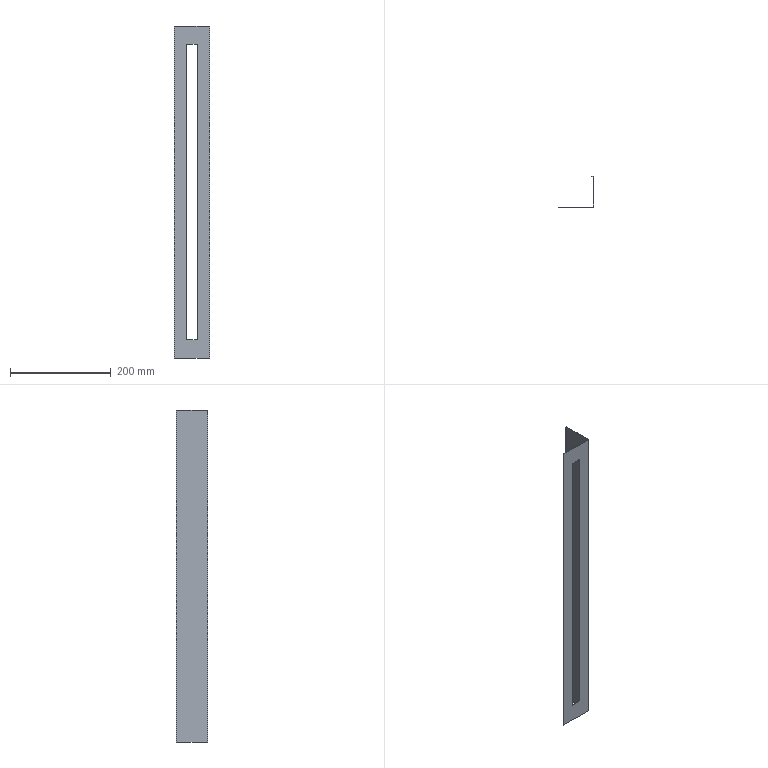Component | SolidWorks | MotorCover-1 | 1 solid | 16 faces | box 70 x 62 x 660 mm | volume 37993 mm3 | plane 14 | cylinder 2 | commonest cylinder face diameters 1 x2
build123d program:
from build123d import *

# Parameters (mm, degrees)
BOSS_EXTRUDE1_DEPTH = 660
SKETCH2_W           = 588
SKETCH2_H           = 21.5
CUT_EXTRUDE1_DEPTH  = 10


with BuildPart() as part:
    # Sketch1 → Boss-Extrude1 (new body)
    with BuildSketch(Plane.XY):
        with BuildLine():
            Line((0, 0), (0, 69.5))
            ThreePointArc((0, 69.5), (0.1464, 69.854), (0.5, 70))
            Line((0.5, 70), (61.5, 70))
            ThreePointArc((61.5, 70), (61.854, 69.854), (62, 69.5))
            Line((62, 69.5), (62, 66.5))
            Line((62, 66.5), (61.5, 66.5))
            Line((61.5, 66.5), (61.5, 69.5))
            Line((61.5, 69.5), (0.5, 69.5))
            Line((0.5, 69.5), (0.5, 0))
            Line((0.5, 0), (0, 0))
        make_face()
    extrude(amount=BOSS_EXTRUDE1_DEPTH)

    # Sketch2 → Cut-Extrude1 (cut)
    with BuildSketch(Plane.ZY):
        with Locations((330, 34.75)):
            Rectangle(SKETCH2_W, SKETCH2_H)
    extrude(amount=-CUT_EXTRUDE1_DEPTH, mode=Mode.SUBTRACT)


solid = part.part

# Placed as in the assembly
solid = solid.moved(Location((-76.793, -54.753, 1606.064), (180, 0, -90)))
STEP:
#1=CARTESIAN_POINT('',(-3.023,-2.156,63.231));
#2=VERTEX_POINT('',#1);
#3=CARTESIAN_POINT('',(-3.023,-2.136,63.231));
#4=VERTEX_POINT('',#3);
#5=CARTESIAN_POINT('',(-3.023,-2.136,63.231));
#6=DIRECTION('',(-0.,1.,0.));
#7=VECTOR('',#6,39.37);
#8=LINE('',#5,#7);
#9=EDGE_CURVE('',#2,#4,#8,.T.);
#10=ORIENTED_EDGE('',*,*,#9,.T.);
#11=CARTESIAN_POINT('',(-3.023,-2.136,37.247));
#12=VERTEX_POINT('',#11);
#13=CARTESIAN_POINT('',(-3.023,-2.136,37.247));
#14=DIRECTION('',(0.,-0.,1.));
#15=VECTOR('',#14,39.37);
#16=LINE('',#13,#15);
#17=EDGE_CURVE('',#12,#4,#16,.T.);
#18=ORIENTED_EDGE('',*,*,#17,.F.);
#19=CARTESIAN_POINT('',(-3.023,-2.156,37.247));
#20=VERTEX_POINT('',#19);
#21=CARTESIAN_POINT('',(-3.023,-2.136,37.247));
#22=DIRECTION('',(-0.,1.,0.));
#23=VECTOR('',#22,39.37);
#24=LINE('',#21,#23);
#25=EDGE_CURVE('',#20,#12,#24,.T.);
#26=ORIENTED_EDGE('',*,*,#25,.F.);
#27=CARTESIAN_POINT('',(-3.023,-2.156,37.247));
#28=DIRECTION('',(0.,-0.,1.));
#29=VECTOR('',#28,39.37);
#30=LINE('',#27,#29);
#31=EDGE_CURVE('',#20,#2,#30,.T.);
#32=ORIENTED_EDGE('',*,*,#31,.T.);
#33=EDGE_LOOP('',(#10,#18,#26,#32));
#34=FACE_OUTER_BOUND('',#33,.T.);
#35=CARTESIAN_POINT('',(-3.023,-2.136,37.247));
#36=DIRECTION('',(1.,0.,-0.));
#37=DIRECTION('',(-0.,0.,-1.));
#38=AXIS2_PLACEMENT_3D('',#35,#36,#37);
#39=PLANE('',#38);
#40=ADVANCED_FACE('',(#34),#39,.F.);
#41=CARTESIAN_POINT('',(-2.078,-2.136,38.664));
#42=VERTEX_POINT('',#41);
#43=CARTESIAN_POINT('',(-1.232,-2.136,38.664));
#44=VERTEX_POINT('',#43);
#45=CARTESIAN_POINT('',(-0.2871,-2.136,38.664));
#46=DIRECTION('',(1.,0.,-0.));
#47=VECTOR('',#46,39.37);
#48=LINE('',#45,#47);
#49=EDGE_CURVE('',#42,#44,#48,.T.);
#50=ORIENTED_EDGE('',*,*,#49,.T.);
#51=CARTESIAN_POINT('',(-1.232,-2.136,61.814));
#52=VERTEX_POINT('',#51);
#53=CARTESIAN_POINT('',(-1.232,-2.136,37.247));
#54=DIRECTION('',(0.,-0.,1.));
#55=VECTOR('',#54,39.37);
#56=LINE('',#53,#55);
#57=EDGE_CURVE('',#44,#52,#56,.T.);
#58=ORIENTED_EDGE('',*,*,#57,.T.);
#59=CARTESIAN_POINT('',(-2.078,-2.136,61.814));
#60=VERTEX_POINT('',#59);
#61=CARTESIAN_POINT('',(-0.2871,-2.136,61.814));
#62=DIRECTION('',(-1.,-0.,0.));
#63=VECTOR('',#62,39.37);
#64=LINE('',#61,#63);
#65=EDGE_CURVE('',#52,#60,#64,.T.);
#66=ORIENTED_EDGE('',*,*,#65,.T.);
#67=CARTESIAN_POINT('',(-2.078,-2.136,37.247));
#68=DIRECTION('',(-0.,0.,-1.));
#69=VECTOR('',#68,39.37);
#70=LINE('',#67,#69);
#71=EDGE_CURVE('',#60,#42,#70,.T.);
#72=ORIENTED_EDGE('',*,*,#71,.T.);
#73=EDGE_LOOP('',(#50,#58,#66,#72));
#74=FACE_BOUND('',#73,.T.);
#75=CARTESIAN_POINT('',(-0.2871,-2.136,63.231));
#76=VERTEX_POINT('',#75);
#77=CARTESIAN_POINT('',(-0.2871,-2.136,63.231));
#78=DIRECTION('',(1.,0.,-0.));
#79=VECTOR('',#78,39.37);
#80=LINE('',#77,#79);
#81=EDGE_CURVE('',#4,#76,#80,.T.);
#82=ORIENTED_EDGE('',*,*,#81,.T.);
#83=CARTESIAN_POINT('',(-0.2871,-2.136,37.247));
#84=VERTEX_POINT('',#83);
#85=CARTESIAN_POINT('',(-0.2871,-2.136,37.247));
#86=DIRECTION('',(0.,-0.,1.));
#87=VECTOR('',#86,39.37);
#88=LINE('',#85,#87);
#89=EDGE_CURVE('',#84,#76,#88,.T.);
#90=ORIENTED_EDGE('',*,*,#89,.F.);
#91=CARTESIAN_POINT('',(-0.2871,-2.136,37.247));
#92=DIRECTION('',(1.,0.,-0.));
#93=VECTOR('',#92,39.37);
#94=LINE('',#91,#93);
#95=EDGE_CURVE('',#12,#84,#94,.T.);
#96=ORIENTED_EDGE('',*,*,#95,.F.);
#97=ORIENTED_EDGE('',*,*,#17,.T.);
#98=EDGE_LOOP('',(#82,#90,#96,#97));
#99=FACE_OUTER_BOUND('',#98,.T.);
#100=CARTESIAN_POINT('',(-0.2871,-2.136,37.247));
#101=DIRECTION('',(0.,-1.,-0.));
#102=DIRECTION('',(-1.,-0.,0.));
#103=AXIS2_PLACEMENT_3D('',#100,#101,#102);
#104=PLANE('',#103);
#105=ADVANCED_FACE('',(#74,#99),#104,.F.);
#106=CARTESIAN_POINT('',(-0.2871,0.2656,63.231));
#107=VERTEX_POINT('',#106);
#108=CARTESIAN_POINT('',(-0.2871,0.2656,63.231));
#109=DIRECTION('',(-0.,1.,0.));
#110=VECTOR('',#109,39.37);
#111=LINE('',#108,#110);
#112=EDGE_CURVE('',#76,#107,#111,.T.);
#113=ORIENTED_EDGE('',*,*,#112,.T.);
#114=CARTESIAN_POINT('',(-0.2871,0.2656,37.247));
#115=VERTEX_POINT('',#114);
#116=CARTESIAN_POINT('',(-0.2871,0.2656,37.247));
#117=DIRECTION('',(0.,-0.,1.));
#118=VECTOR('',#117,39.37);
#119=LINE('',#116,#118);
#120=EDGE_CURVE('',#115,#107,#119,.T.);
#121=ORIENTED_EDGE('',*,*,#120,.F.);
#122=CARTESIAN_POINT('',(-0.2871,0.2656,37.247));
#123=DIRECTION('',(-0.,1.,0.));
#124=VECTOR('',#123,39.37);
#125=LINE('',#122,#124);
#126=EDGE_CURVE('',#84,#115,#125,.T.);
#127=ORIENTED_EDGE('',*,*,#126,.F.);
#128=ORIENTED_EDGE('',*,*,#89,.T.);
#129=EDGE_LOOP('',(#113,#121,#127,#128));
#130=FACE_OUTER_BOUND('',#129,.T.);
#131=CARTESIAN_POINT('',(-0.2871,0.2656,37.247));
#132=DIRECTION('',(1.,0.,-0.));
#133=DIRECTION('',(-0.,0.,-1.));
#134=AXIS2_PLACEMENT_3D('',#131,#132,#133);
#135=PLANE('',#134);
#136=ADVANCED_FACE('',(#130),#135,.F.);
#137=CARTESIAN_POINT('',(-0.4053,0.2656,63.231));
#138=VERTEX_POINT('',#137);
#139=CARTESIAN_POINT('',(-0.4053,0.2656,63.231));
#140=DIRECTION('',(-1.,-0.,0.));
#141=VECTOR('',#140,39.37);
#142=LINE('',#139,#141);
#143=EDGE_CURVE('',#107,#138,#142,.T.);
#144=ORIENTED_EDGE('',*,*,#143,.T.);
#145=CARTESIAN_POINT('',(-0.4053,0.2656,37.247));
#146=VERTEX_POINT('',#145);
#147=CARTESIAN_POINT('',(-0.4053,0.2656,37.247));
#148=DIRECTION('',(0.,-0.,1.));
#149=VECTOR('',#148,39.37);
#150=LINE('',#147,#149);
#151=EDGE_CURVE('',#146,#138,#150,.T.);
#152=ORIENTED_EDGE('',*,*,#151,.F.);
#153=CARTESIAN_POINT('',(-0.4053,0.2656,37.247));
#154=DIRECTION('',(-1.,-0.,0.));
#155=VECTOR('',#154,39.37);
#156=LINE('',#153,#155);
#157=EDGE_CURVE('',#115,#146,#156,.T.);
#158=ORIENTED_EDGE('',*,*,#157,.F.);
#159=ORIENTED_EDGE('',*,*,#120,.T.);
#160=EDGE_LOOP('',(#144,#152,#158,#159));
#161=FACE_OUTER_BOUND('',#160,.T.);
#162=CARTESIAN_POINT('',(-0.4053,0.2656,37.247));
#163=DIRECTION('',(-0.,1.,0.));
#164=DIRECTION('',(0.,-0.,1.));
#165=AXIS2_PLACEMENT_3D('',#162,#163,#164);
#166=PLANE('',#165);
#167=ADVANCED_FACE('',(#161),#166,.F.);
#168=CARTESIAN_POINT('',(-0.4053,0.2853,63.231));
#169=VERTEX_POINT('',#168);
#170=CARTESIAN_POINT('',(-0.4053,0.2853,63.231));
#171=DIRECTION('',(-0.,1.,0.));
#172=VECTOR('',#171,39.37);
#173=LINE('',#170,#172);
#174=EDGE_CURVE('',#138,#169,#173,.T.);
#175=ORIENTED_EDGE('',*,*,#174,.T.);
#176=CARTESIAN_POINT('',(-0.4053,0.2853,37.247));
#177=VERTEX_POINT('',#176);
#178=CARTESIAN_POINT('',(-0.4053,0.2853,37.247));
#179=DIRECTION('',(0.,-0.,1.));
#180=VECTOR('',#179,39.37);
#181=LINE('',#178,#180);
#182=EDGE_CURVE('',#177,#169,#181,.T.);
#183=ORIENTED_EDGE('',*,*,#182,.F.);
#184=CARTESIAN_POINT('',(-0.4053,0.2853,37.247));
#185=DIRECTION('',(-0.,1.,0.));
#186=VECTOR('',#185,39.37);
#187=LINE('',#184,#186);
#188=EDGE_CURVE('',#146,#177,#187,.T.);
#189=ORIENTED_EDGE('',*,*,#188,.F.);
#190=ORIENTED_EDGE('',*,*,#151,.T.);
#191=EDGE_LOOP('',(#175,#183,#189,#190));
#192=FACE_OUTER_BOUND('',#191,.T.);
#193=CARTESIAN_POINT('',(-0.4053,0.2853,37.247));
#194=DIRECTION('',(1.,0.,-0.));
#195=DIRECTION('',(-0.,0.,-1.));
#196=AXIS2_PLACEMENT_3D('',#193,#194,#195);
#197=PLANE('',#196);
#198=ADVANCED_FACE('',(#192),#197,.F.);
#199=CARTESIAN_POINT('',(-0.2871,0.2853,63.231));
#200=VERTEX_POINT('',#199);
#201=CARTESIAN_POINT('',(-0.2871,0.2853,63.231));
#202=DIRECTION('',(1.,0.,-0.));
#203=VECTOR('',#202,39.37);
#204=LINE('',#201,#203);
#205=EDGE_CURVE('',#169,#200,#204,.T.);
#206=ORIENTED_EDGE('',*,*,#205,.T.);
#207=CARTESIAN_POINT('',(-0.2871,0.2853,37.247));
#208=VERTEX_POINT('',#207);
#209=CARTESIAN_POINT('',(-0.2871,0.2853,37.247));
#210=DIRECTION('',(0.,-0.,1.));
#211=VECTOR('',#210,39.37);
#212=LINE('',#209,#211);
#213=EDGE_CURVE('',#208,#200,#212,.T.);
#214=ORIENTED_EDGE('',*,*,#213,.F.);
#215=CARTESIAN_POINT('',(-0.2871,0.2853,37.247));
#216=DIRECTION('',(1.,0.,-0.));
#217=VECTOR('',#216,39.37);
#218=LINE('',#215,#217);
#219=EDGE_CURVE('',#177,#208,#218,.T.);
#220=ORIENTED_EDGE('',*,*,#219,.F.);
#221=ORIENTED_EDGE('',*,*,#182,.T.);
#222=EDGE_LOOP('',(#206,#214,#220,#221));
#223=FACE_OUTER_BOUND('',#222,.T.);
#224=CARTESIAN_POINT('',(-0.2871,0.2853,37.247));
#225=DIRECTION('',(0.,-1.,-0.));
#226=DIRECTION('',(-0.,0.,-1.));
#227=AXIS2_PLACEMENT_3D('',#224,#225,#226);
#228=PLANE('',#227);
#229=ADVANCED_FACE('',(#223),#228,.F.);
#230=CARTESIAN_POINT('',(-0.2675,0.2656,63.231));
#231=VERTEX_POINT('',#230);
#232=CARTESIAN_POINT('',(-0.2871,0.2656,63.231));
#233=DIRECTION('',(-0.,0.,-1.));
#234=DIRECTION('',(0.,-1.,0.));
#235=AXIS2_PLACEMENT_3D('',#232,#233,#234);
#236=CIRCLE('',#235,0.01969);
#237=EDGE_CURVE('',#200,#231,#236,.T.);
#238=ORIENTED_EDGE('',*,*,#237,.T.);
#239=CARTESIAN_POINT('',(-0.2675,0.2656,37.247));
#240=VERTEX_POINT('',#239);
#241=CARTESIAN_POINT('',(-0.2675,0.2656,37.247));
#242=DIRECTION('',(0.,-0.,1.));
#243=VECTOR('',#242,39.37);
#244=LINE('',#241,#243);
#245=EDGE_CURVE('',#240,#231,#244,.T.);
#246=ORIENTED_EDGE('',*,*,#245,.F.);
#247=CARTESIAN_POINT('',(-0.2871,0.2656,37.247));
#248=DIRECTION('',(-0.,0.,-1.));
#249=DIRECTION('',(0.,-1.,0.));
#250=AXIS2_PLACEMENT_3D('',#247,#248,#249);
#251=CIRCLE('',#250,0.01969);
#252=EDGE_CURVE('',#208,#240,#251,.T.);
#253=ORIENTED_EDGE('',*,*,#252,.F.);
#254=ORIENTED_EDGE('',*,*,#213,.T.);
#255=EDGE_LOOP('',(#238,#246,#253,#254));
#256=FACE_OUTER_BOUND('',#255,.T.);
#257=CARTESIAN_POINT('',(-0.2871,0.2656,37.247));
#258=DIRECTION('',(0.,-0.,1.));
#259=DIRECTION('',(0.,-1.,0.));
#260=AXIS2_PLACEMENT_3D('',#257,#258,#259);
#261=CYLINDRICAL_SURFACE('',#260,0.01969);
#262=ADVANCED_FACE('',(#256),#261,.T.);
#263=CARTESIAN_POINT('',(-0.2675,-2.136,63.231));
#264=VERTEX_POINT('',#263);
#265=CARTESIAN_POINT('',(-0.2675,-2.136,63.231));
#266=DIRECTION('',(0.,-1.,-0.));
#267=VECTOR('',#266,39.37);
#268=LINE('',#265,#267);
#269=EDGE_CURVE('',#231,#264,#268,.T.);
#270=ORIENTED_EDGE('',*,*,#269,.T.);
#271=CARTESIAN_POINT('',(-0.2675,-2.136,37.247));
#272=VERTEX_POINT('',#271);
#273=CARTESIAN_POINT('',(-0.2675,-2.136,37.247));
#274=DIRECTION('',(0.,-0.,1.));
#275=VECTOR('',#274,39.37);
#276=LINE('',#273,#275);
#277=EDGE_CURVE('',#272,#264,#276,.T.);
#278=ORIENTED_EDGE('',*,*,#277,.F.);
#279=CARTESIAN_POINT('',(-0.2675,-2.136,37.247));
#280=DIRECTION('',(0.,-1.,-0.));
#281=VECTOR('',#280,39.37);
#282=LINE('',#279,#281);
#283=EDGE_CURVE('',#240,#272,#282,.T.);
#284=ORIENTED_EDGE('',*,*,#283,.F.);
#285=ORIENTED_EDGE('',*,*,#245,.T.);
#286=EDGE_LOOP('',(#270,#278,#284,#285));
#287=FACE_OUTER_BOUND('',#286,.T.);
#288=CARTESIAN_POINT('',(-0.2675,-2.136,37.247));
#289=DIRECTION('',(-1.,-0.,0.));
#290=DIRECTION('',(0.,-0.,1.));
#291=AXIS2_PLACEMENT_3D('',#288,#289,#290);
#292=PLANE('',#291);
#293=ADVANCED_FACE('',(#287),#292,.F.);
#294=CARTESIAN_POINT('',(-0.2871,-2.156,63.231));
#295=VERTEX_POINT('',#294);
#296=CARTESIAN_POINT('',(-0.2871,-2.136,63.231));
#297=DIRECTION('',(-0.,0.,-1.));
#298=DIRECTION('',(0.,-1.,0.));
#299=AXIS2_PLACEMENT_3D('',#296,#297,#298);
#300=CIRCLE('',#299,0.01969);
#301=EDGE_CURVE('',#264,#295,#300,.T.);
#302=ORIENTED_EDGE('',*,*,#301,.T.);
#303=CARTESIAN_POINT('',(-0.2871,-2.156,37.247));
#304=VERTEX_POINT('',#303);
#305=CARTESIAN_POINT('',(-0.2871,-2.156,37.247));
#306=DIRECTION('',(0.,-0.,1.));
#307=VECTOR('',#306,39.37);
#308=LINE('',#305,#307);
#309=EDGE_CURVE('',#304,#295,#308,.T.);
#310=ORIENTED_EDGE('',*,*,#309,.F.);
#311=CARTESIAN_POINT('',(-0.2871,-2.136,37.247));
#312=DIRECTION('',(-0.,0.,-1.));
#313=DIRECTION('',(0.,-1.,0.));
#314=AXIS2_PLACEMENT_3D('',#311,#312,#313);
#315=CIRCLE('',#314,0.01969);
#316=EDGE_CURVE('',#272,#304,#315,.T.);
#317=ORIENTED_EDGE('',*,*,#316,.F.);
#318=ORIENTED_EDGE('',*,*,#277,.T.);
#319=EDGE_LOOP('',(#302,#310,#317,#318));
#320=FACE_OUTER_BOUND('',#319,.T.);
#321=CARTESIAN_POINT('',(-0.2871,-2.136,37.247));
#322=DIRECTION('',(0.,-0.,1.));
#323=DIRECTION('',(0.,-1.,0.));
#324=AXIS2_PLACEMENT_3D('',#321,#322,#323);
#325=CYLINDRICAL_SURFACE('',#324,0.01969);
#326=ADVANCED_FACE('',(#320),#325,.T.);
#327=CARTESIAN_POINT('',(-1.232,-2.156,61.814));
#328=VERTEX_POINT('',#327);
#329=CARTESIAN_POINT('',(-2.078,-2.156,61.814));
#330=VERTEX_POINT('',#329);
#331=CARTESIAN_POINT('',(-1.232,-2.156,61.814));
#332=DIRECTION('',(-1.,-0.,0.));
#333=VECTOR('',#332,39.37);
#334=LINE('',#331,#333);
#335=EDGE_CURVE('',#328,#330,#334,.T.);
#336=ORIENTED_EDGE('',*,*,#335,.F.);
#337=CARTESIAN_POINT('',(-1.232,-2.156,38.664));
#338=VERTEX_POINT('',#337);
#339=CARTESIAN_POINT('',(-1.232,-2.156,38.664));
#340=DIRECTION('',(0.,-0.,1.));
#341=VECTOR('',#340,39.37);
#342=LINE('',#339,#341);
#343=EDGE_CURVE('',#338,#328,#342,.T.);
#344=ORIENTED_EDGE('',*,*,#343,.F.);
#345=CARTESIAN_POINT('',(-2.078,-2.156,38.664));
#346=VERTEX_POINT('',#345);
#347=CARTESIAN_POINT('',(-2.078,-2.156,38.664));
#348=DIRECTION('',(1.,0.,-0.));
#349=VECTOR('',#348,39.37);
#350=LINE('',#347,#349);
#351=EDGE_CURVE('',#346,#338,#350,.T.);
#352=ORIENTED_EDGE('',*,*,#351,.F.);
#353=CARTESIAN_POINT('',(-2.078,-2.156,61.814));
#354=DIRECTION('',(-0.,0.,-1.));
#355=VECTOR('',#354,39.37);
#356=LINE('',#353,#355);
#357=EDGE_CURVE('',#330,#346,#356,.T.);
#358=ORIENTED_EDGE('',*,*,#357,.F.);
#359=EDGE_LOOP('',(#336,#344,#352,#358));
#360=FACE_BOUND('',#359,.T.);
#361=CARTESIAN_POINT('',(-3.023,-2.156,63.231));
#362=DIRECTION('',(-1.,-0.,0.));
#363=VECTOR('',#362,39.37);
#364=LINE('',#361,#363);
#365=EDGE_CURVE('',#295,#2,#364,.T.);
#366=ORIENTED_EDGE('',*,*,#365,.T.);
#367=ORIENTED_EDGE('',*,*,#31,.F.);
#368=CARTESIAN_POINT('',(-3.023,-2.156,37.247));
#369=DIRECTION('',(-1.,-0.,0.));
#370=VECTOR('',#369,39.37);
#371=LINE('',#368,#370);
#372=EDGE_CURVE('',#304,#20,#371,.T.);
#373=ORIENTED_EDGE('',*,*,#372,.F.);
#374=ORIENTED_EDGE('',*,*,#309,.T.);
#375=EDGE_LOOP('',(#366,#367,#373,#374));
#376=FACE_OUTER_BOUND('',#375,.T.);
#377=CARTESIAN_POINT('',(-3.023,-2.156,37.247));
#378=DIRECTION('',(-0.,1.,0.));
#379=DIRECTION('',(0.,-0.,1.));
#380=AXIS2_PLACEMENT_3D('',#377,#378,#379);
#381=PLANE('',#380);
#382=ADVANCED_FACE('',(#360,#376),#381,.F.);
#383=ORIENTED_EDGE('',*,*,#25,.T.);
#384=ORIENTED_EDGE('',*,*,#95,.T.);
#385=ORIENTED_EDGE('',*,*,#126,.T.);
#386=ORIENTED_EDGE('',*,*,#157,.T.);
#387=ORIENTED_EDGE('',*,*,#188,.T.);
#388=ORIENTED_EDGE('',*,*,#219,.T.);
#389=ORIENTED_EDGE('',*,*,#252,.T.);
#390=ORIENTED_EDGE('',*,*,#283,.T.);
#391=ORIENTED_EDGE('',*,*,#316,.T.);
#392=ORIENTED_EDGE('',*,*,#372,.T.);
#393=EDGE_LOOP('',(#383,#384,#385,#386,#387,#388,#389,#390,#391,#392));
#394=FACE_OUTER_BOUND('',#393,.T.);
#395=CARTESIAN_POINT('',(-0.2871,-2.136,37.247));
#396=DIRECTION('',(0.,-0.,1.));
#397=DIRECTION('',(0.,-1.,-0.));
#398=AXIS2_PLACEMENT_3D('',#395,#396,#397);
#399=PLANE('',#398);
#400=ADVANCED_FACE('',(#394),#399,.F.);
#401=ORIENTED_EDGE('',*,*,#9,.F.);
#402=ORIENTED_EDGE('',*,*,#365,.F.);
#403=ORIENTED_EDGE('',*,*,#301,.F.);
#404=ORIENTED_EDGE('',*,*,#269,.F.);
#405=ORIENTED_EDGE('',*,*,#237,.F.);
#406=ORIENTED_EDGE('',*,*,#205,.F.);
#407=ORIENTED_EDGE('',*,*,#174,.F.);
#408=ORIENTED_EDGE('',*,*,#143,.F.);
#409=ORIENTED_EDGE('',*,*,#112,.F.);
#410=ORIENTED_EDGE('',*,*,#81,.F.);
#411=EDGE_LOOP('',(#401,#402,#403,#404,#405,#406,#407,#408,#409,#410));
#412=FACE_OUTER_BOUND('',#411,.T.);
#413=CARTESIAN_POINT('',(-0.2871,-2.136,63.231));
#414=DIRECTION('',(0.,-0.,1.));
#415=DIRECTION('',(0.,-1.,-0.));
#416=AXIS2_PLACEMENT_3D('',#413,#414,#415);
#417=PLANE('',#416);
#418=ADVANCED_FACE('',(#412),#417,.T.);
#419=CARTESIAN_POINT('',(-1.232,-1.762,38.664));
#420=DIRECTION('',(0.,-1.,-0.));
#421=VECTOR('',#420,39.37);
#422=LINE('',#419,#421);
#423=EDGE_CURVE('',#44,#338,#422,.T.);
#424=ORIENTED_EDGE('',*,*,#423,.T.);
#425=ORIENTED_EDGE('',*,*,#343,.T.);
#426=CARTESIAN_POINT('',(-1.232,-1.762,61.814));
#427=DIRECTION('',(0.,-1.,-0.));
#428=VECTOR('',#427,39.37);
#429=LINE('',#426,#428);
#430=EDGE_CURVE('',#52,#328,#429,.T.);
#431=ORIENTED_EDGE('',*,*,#430,.F.);
#432=ORIENTED_EDGE('',*,*,#57,.F.);
#433=EDGE_LOOP('',(#424,#425,#431,#432));
#434=FACE_OUTER_BOUND('',#433,.T.);
#435=CARTESIAN_POINT('',(-1.232,-1.762,38.664));
#436=DIRECTION('',(1.,0.,-0.));
#437=DIRECTION('',(-0.,0.,-1.));
#438=AXIS2_PLACEMENT_3D('',#435,#436,#437);
#439=PLANE('',#438);
#440=ADVANCED_FACE('',(#434),#439,.F.);
#441=CARTESIAN_POINT('',(-2.078,-1.762,38.664));
#442=DIRECTION('',(0.,-1.,-0.));
#443=VECTOR('',#442,39.37);
#444=LINE('',#441,#443);
#445=EDGE_CURVE('',#42,#346,#444,.T.);
#446=ORIENTED_EDGE('',*,*,#445,.T.);
#447=ORIENTED_EDGE('',*,*,#351,.T.);
#448=ORIENTED_EDGE('',*,*,#423,.F.);
#449=ORIENTED_EDGE('',*,*,#49,.F.);
#450=EDGE_LOOP('',(#446,#447,#448,#449));
#451=FACE_OUTER_BOUND('',#450,.T.);
#452=CARTESIAN_POINT('',(-2.078,-1.762,38.664));
#453=DIRECTION('',(-0.,0.,-1.));
#454=DIRECTION('',(-0.,1.,0.));
#455=AXIS2_PLACEMENT_3D('',#452,#453,#454);
#456=PLANE('',#455);
#457=ADVANCED_FACE('',(#451),#456,.F.);
#458=CARTESIAN_POINT('',(-2.078,-1.762,61.814));
#459=DIRECTION('',(0.,-1.,-0.));
#460=VECTOR('',#459,39.37);
#461=LINE('',#458,#460);
#462=EDGE_CURVE('',#60,#330,#461,.T.);
#463=ORIENTED_EDGE('',*,*,#462,.T.);
#464=ORIENTED_EDGE('',*,*,#357,.T.);
#465=ORIENTED_EDGE('',*,*,#445,.F.);
#466=ORIENTED_EDGE('',*,*,#71,.F.);
#467=EDGE_LOOP('',(#463,#464,#465,#466));
#468=FACE_OUTER_BOUND('',#467,.T.);
#469=CARTESIAN_POINT('',(-2.078,-1.762,61.814));
#470=DIRECTION('',(-1.,-0.,0.));
#471=DIRECTION('',(0.,-0.,1.));
#472=AXIS2_PLACEMENT_3D('',#469,#470,#471);
#473=PLANE('',#472);
#474=ADVANCED_FACE('',(#468),#473,.F.);
#475=ORIENTED_EDGE('',*,*,#430,.T.);
#476=ORIENTED_EDGE('',*,*,#335,.T.);
#477=ORIENTED_EDGE('',*,*,#462,.F.);
#478=ORIENTED_EDGE('',*,*,#65,.F.);
#479=EDGE_LOOP('',(#475,#476,#477,#478));
#480=FACE_OUTER_BOUND('',#479,.T.);
#481=CARTESIAN_POINT('',(-1.232,-1.762,61.814));
#482=DIRECTION('',(0.,-0.,1.));
#483=DIRECTION('',(1.,0.,-0.));
#484=AXIS2_PLACEMENT_3D('',#481,#482,#483);
#485=PLANE('',#484);
#486=ADVANCED_FACE('',(#480),#485,.F.);
#487=CLOSED_SHELL('',(#40,#105,#136,#167,#198,#229,#262,#293,#326,#382,#400,#418,#440,#457,#474,#486));
#488=MANIFOLD_SOLID_BREP('',#487);
#489=CARTESIAN_POINT('',(0.,0.,0.));
#490=DIRECTION('',(0.,0.,1.));
#491=DIRECTION('',(1.,0.,0.));
#492=AXIS2_PLACEMENT_3D('',#489,#490,#491);
#493=(LENGTH_UNIT()NAMED_UNIT(*)SI_UNIT($,.METRE.));
#494=LENGTH_MEASURE_WITH_UNIT(LENGTH_MEASURE(0.0254),#493);
#495=DIMENSIONAL_EXPONENTS(1.,0.,0.,0.,0.,0.,0.);
#496=(CONVERSION_BASED_UNIT('',#494)LENGTH_UNIT()NAMED_UNIT(#495));
#497=UNCERTAINTY_MEASURE_WITH_UNIT(LENGTH_MEASURE(0.00001),#496,'','');
#498=(NAMED_UNIT(*)PLANE_ANGLE_UNIT()SI_UNIT($,.RADIAN.));
#499=(NAMED_UNIT(*)SI_UNIT($,.STERADIAN.)SOLID_ANGLE_UNIT());
#500=(GEOMETRIC_REPRESENTATION_CONTEXT(3)GLOBAL_UNCERTAINTY_ASSIGNED_CONTEXT((#497))GLOBAL_UNIT_ASSIGNED_CONTEXT((#496,#498,#499))REPRESENTATION_CONTEXT('',''));
#501=ADVANCED_BREP_SHAPE_REPRESENTATION('',(#488,#492),#500);
#502=COLOUR_RGB('',0.7922,0.8196,0.9333);
#503=FILL_AREA_STYLE_COLOUR('',#502);
#504=FILL_AREA_STYLE('',(#503));
#505=SURFACE_STYLE_FILL_AREA(#504);
#506=SURFACE_SIDE_STYLE('',(#505));
#507=SURFACE_STYLE_USAGE(.BOTH.,#506);
#508=PRESENTATION_STYLE_ASSIGNMENT((#507));
#509=STYLED_ITEM('',(#508),#488);
#510=(LENGTH_UNIT()NAMED_UNIT(*)SI_UNIT($,.METRE.));
#511=LENGTH_MEASURE_WITH_UNIT(LENGTH_MEASURE(0.0254),#510);
#512=DIMENSIONAL_EXPONENTS(1.,0.,0.,0.,0.,0.,0.);
#513=(CONVERSION_BASED_UNIT('',#511)LENGTH_UNIT()NAMED_UNIT(#512));
#514=UNCERTAINTY_MEASURE_WITH_UNIT(LENGTH_MEASURE(0.00001),#513,'','');
#515=(NAMED_UNIT(*)PLANE_ANGLE_UNIT()SI_UNIT($,.RADIAN.));
#516=(NAMED_UNIT(*)SI_UNIT($,.STERADIAN.)SOLID_ANGLE_UNIT());
#517=(GEOMETRIC_REPRESENTATION_CONTEXT(3)GLOBAL_UNCERTAINTY_ASSIGNED_CONTEXT((#514))GLOBAL_UNIT_ASSIGNED_CONTEXT((#513,#515,#516))REPRESENTATION_CONTEXT('',''));
#518=MECHANICAL_DESIGN_GEOMETRIC_PRESENTATION_REPRESENTATION('',(#509),#517);
#519=PRESENTATION_LAYER_ASSIGNMENT('','',(#509));